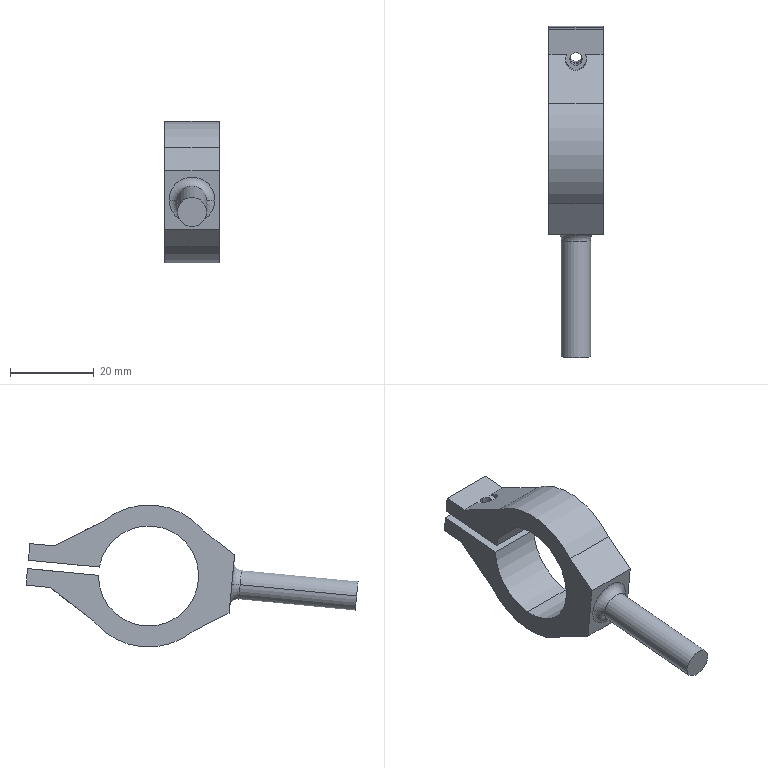Component | SolidWorks | Sleeve(Modified)-1 | 1 solid | 31 faces | box 13 x 79.45 x 34 mm | volume 9617 mm3 | cylinder 15 | plane 14 | torus 2 | commonest cylinder face diameters 3 x4 5 x3 34 x3 24 x3 7 x2 | material Plain Carbon Steel
build123d program:
from build123d import *

# Parameters (mm, degrees)
BOSS_EXTRUDE1_DEPTH      = 6.5
BOSS_EXTRUDE1_DEPTH_BACK = 6.5
SKETCH2_R                = 1.5
CUT_EXTRUDE1_DEPTH       = 37.976
SKETCH3_R                = 3.5
BOSS_EXTRUDE2_DEPTH      = 30
FILLET3_R                = 2
SKETCH4_R                = 2.5
CUT_EXTRUDE2_DEPTH       = 10


with BuildPart() as part:
    # Sketch1 → Boss-Extrude1 (new, two sides: drawn at the far end of the back side and taken through both)
    with BuildSketch(Plane.XY.offset(-BOSS_EXTRUDE1_DEPTH_BACK)):
        with BuildLine():
            Line((-1, 11.958), (-1, 29))
            Line((-1, 29), (-5, 29))
            Line((-5, 29), (-5, 23.19))
            Line((-5, 23.19), (-11.97, 12.071))
            ThreePointArc((-11.97, 12.071), (-17, 0), (-11.97, -12.071))
            Line((-11.97, -12.071), (-7, -20))
            Line((-7, -20), (7, -20))
            Line((7, -20), (11.97, -12.071))
            ThreePointArc((11.97, -12.071), (17, 0), (11.97, 12.071))
            Line((11.97, 12.071), (5, 23.19))
            Line((5, 23.19), (5, 29))
            Line((5, 29), (1, 29))
            Line((1, 29), (1, 11.958))
            ThreePointArc((1, 11.958), (0, -12), (-1, 11.958))
        make_face()
    extrude(amount=BOSS_EXTRUDE1_DEPTH + BOSS_EXTRUDE1_DEPTH_BACK)

    # Sketch2 → Cut-Extrude1 (cut, through all)
    with BuildSketch(Plane.ZY.offset(5)):
        with Locations(Location((0, 22, 0), (0, 0, 270))):
            Circle(SKETCH2_R)
    extrude(amount=-CUT_EXTRUDE1_DEPTH, mode=Mode.SUBTRACT)

    # Sketch3 → Boss-Extrude2 (add)
    with BuildSketch(Plane.XZ.offset(20)):
        with Locations(Location((0, 0, 0), (0, 0, 270))):
            Circle(SKETCH3_R)
    extrude(amount=BOSS_EXTRUDE2_DEPTH)

    # Fillet3
    fillet3_edges = [part.edges().sort_by_distance(p)[0] for p in [
        (0, -20, 3.5),
    ]]
    fillet(fillet3_edges, radius=FILLET3_R)

    # Sketch4 → Cut-Extrude2 (cut)
    with BuildSketch(Plane.ZY.offset(5)):
        with Locations((0, 22)):
            Circle(SKETCH4_R)
    cut_extrude2 = extrude(amount=CUT_EXTRUDE2_DEPTH, mode=Mode.SUBTRACT)

    # Mirror1: Cut-Extrude2 across plane
    add(cut_extrude2.mirror(Plane(origin=(0, 0, 0), x_dir=(0, 0, 1), z_dir=(1, 0, 0))), mode=Mode.SUBTRACT)


solid = part.part

# Placed as in the assembly
solid = solid.moved(Location((182.562, 15.115, 349), (5.48, -90, 0)))
STEP:
#1=CARTESIAN_POINT('',(7.274,1.523,13.631));
#2=VERTEX_POINT('',#1);
#3=CARTESIAN_POINT('',(7.187,1.387,13.527));
#4=VERTEX_POINT('',#3);
#5=CARTESIAN_POINT('',(7.274,1.523,13.631));
#6=CARTESIAN_POINT('',(7.314,1.454,13.579));
#7=CARTESIAN_POINT('',(7.271,1.387,13.527));
#8=CARTESIAN_POINT('',(7.187,1.387,13.527));
#9=(BOUNDED_CURVE()B_SPLINE_CURVE(3,(#5,#6,#7,#8),.UNSPECIFIED.,.F.,.F.)B_SPLINE_CURVE_WITH_KNOTS((4,4),(1.074,3.142),.UNSPECIFIED.)CURVE()GEOMETRIC_REPRESENTATION_ITEM()RATIONAL_B_SPLINE_CURVE((1.,0.6745,0.6745,1.))REPRESENTATION_ITEM(''));
#10=EDGE_CURVE('',#2,#4,#9,.T.);
#11=ORIENTED_EDGE('',*,*,#10,.T.);
#12=CARTESIAN_POINT('',(7.187,1.378,13.618));
#13=VERTEX_POINT('',#12);
#14=CARTESIAN_POINT('',(7.187,1.416,13.226));
#15=DIRECTION('',(0.,-0.09551,0.9954));
#16=VECTOR('',#15,39.37);
#17=LINE('',#14,#16);
#18=EDGE_CURVE('',#4,#13,#17,.T.);
#19=ORIENTED_EDGE('',*,*,#18,.T.);
#20=CARTESIAN_POINT('',(7.187,1.476,13.627));
#21=DIRECTION('',(0.,-0.09551,0.9954));
#22=DIRECTION('',(0.,-0.9954,-0.09551));
#23=AXIS2_PLACEMENT_3D('',#20,#21,#22);
#24=CIRCLE('',#23,0.09843);
#25=EDGE_CURVE('',#13,#2,#24,.T.);
#26=ORIENTED_EDGE('',*,*,#25,.T.);
#27=EDGE_LOOP('',(#11,#19,#26));
#28=FACE_OUTER_BOUND('',#27,.T.);
#29=CARTESIAN_POINT('',(7.187,1.514,13.235));
#30=DIRECTION('',(0.,-0.09551,0.9954));
#31=DIRECTION('',(0.,-0.9954,-0.09551));
#32=AXIS2_PLACEMENT_3D('',#29,#30,#31);
#33=CYLINDRICAL_SURFACE('',#32,0.09843);
#34=ADVANCED_FACE('',(#28),#33,.F.);
#35=CARTESIAN_POINT('',(7.05,-1.364,13.552));
#36=VERTEX_POINT('',#35);
#37=CARTESIAN_POINT('',(7.325,-1.364,13.552));
#38=VERTEX_POINT('',#37);
#39=CARTESIAN_POINT('',(7.187,-1.364,13.552));
#40=DIRECTION('',(0.,-0.9954,-0.09551));
#41=DIRECTION('',(-1.,0.,0.));
#42=AXIS2_PLACEMENT_3D('',#39,#40,#41);
#43=CIRCLE('',#42,0.1378);
#44=EDGE_CURVE('',#36,#38,#43,.T.);
#45=ORIENTED_EDGE('',*,*,#44,.F.);
#46=CARTESIAN_POINT('',(7.05,-0.2671,13.657));
#47=VERTEX_POINT('',#46);
#48=CARTESIAN_POINT('',(7.05,-1.364,13.552));
#49=DIRECTION('',(0.,0.9954,0.09551));
#50=VECTOR('',#49,39.37);
#51=LINE('',#48,#50);
#52=EDGE_CURVE('',#36,#47,#51,.T.);
#53=ORIENTED_EDGE('',*,*,#52,.T.);
#54=CARTESIAN_POINT('',(7.325,-0.2671,13.657));
#55=VERTEX_POINT('',#54);
#56=CARTESIAN_POINT('',(7.187,-0.2671,13.657));
#57=DIRECTION('',(0.,-0.9954,-0.09551));
#58=DIRECTION('',(-1.,0.,0.));
#59=AXIS2_PLACEMENT_3D('',#56,#57,#58);
#60=CIRCLE('',#59,0.1378);
#61=EDGE_CURVE('',#47,#55,#60,.T.);
#62=ORIENTED_EDGE('',*,*,#61,.T.);
#63=CARTESIAN_POINT('',(7.325,-1.364,13.552));
#64=DIRECTION('',(0.,0.9954,0.09551));
#65=VECTOR('',#64,39.37);
#66=LINE('',#63,#65);
#67=EDGE_CURVE('',#38,#55,#66,.T.);
#68=ORIENTED_EDGE('',*,*,#67,.F.);
#69=EDGE_LOOP('',(#45,#53,#62,#68));
#70=FACE_OUTER_BOUND('',#69,.T.);
#71=CARTESIAN_POINT('',(7.187,-1.364,13.552));
#72=DIRECTION('',(0.,0.9954,0.09551));
#73=DIRECTION('',(1.,0.,0.));
#74=AXIS2_PLACEMENT_3D('',#71,#72,#73);
#75=CYLINDRICAL_SURFACE('',#74,0.1378);
#76=ADVANCED_FACE('',(#70),#75,.T.);
#77=CARTESIAN_POINT('',(7.187,1.395,13.856));
#78=VERTEX_POINT('',#77);
#79=CARTESIAN_POINT('',(7.187,1.512,13.868));
#80=VERTEX_POINT('',#79);
#81=CARTESIAN_POINT('',(7.187,1.454,13.862));
#82=DIRECTION('',(0.,0.09551,-0.9954));
#83=DIRECTION('',(0.,0.9954,0.09551));
#84=AXIS2_PLACEMENT_3D('',#81,#82,#83);
#85=CIRCLE('',#84,0.05906);
#86=EDGE_CURVE('',#78,#80,#85,.T.);
#87=ORIENTED_EDGE('',*,*,#86,.T.);
#88=CARTESIAN_POINT('',(7.187,1.497,14.024));
#89=VERTEX_POINT('',#88);
#90=CARTESIAN_POINT('',(7.187,1.58,13.162));
#91=DIRECTION('',(0.,-0.09551,0.9954));
#92=VECTOR('',#91,39.37);
#93=LINE('',#90,#92);
#94=EDGE_CURVE('',#80,#89,#93,.T.);
#95=ORIENTED_EDGE('',*,*,#94,.T.);
#96=CARTESIAN_POINT('',(7.187,1.38,14.013));
#97=VERTEX_POINT('',#96);
#98=CARTESIAN_POINT('',(7.187,1.438,14.019));
#99=DIRECTION('',(0.,-0.09551,0.9954));
#100=DIRECTION('',(0.,-0.9954,-0.09551));
#101=AXIS2_PLACEMENT_3D('',#98,#99,#100);
#102=CIRCLE('',#101,0.05906);
#103=EDGE_CURVE('',#89,#97,#102,.T.);
#104=ORIENTED_EDGE('',*,*,#103,.T.);
#105=CARTESIAN_POINT('',(7.187,1.462,13.151));
#106=DIRECTION('',(0.,-0.09551,0.9954));
#107=VECTOR('',#106,39.37);
#108=LINE('',#105,#107);
#109=EDGE_CURVE('',#78,#97,#108,.T.);
#110=ORIENTED_EDGE('',*,*,#109,.F.);
#111=EDGE_LOOP('',(#87,#95,#104,#110));
#112=FACE_OUTER_BOUND('',#111,.T.);
#113=CARTESIAN_POINT('',(7.187,1.521,13.157));
#114=DIRECTION('',(0.,-0.09551,0.9954));
#115=DIRECTION('',(0.,-0.9954,-0.09551));
#116=AXIS2_PLACEMENT_3D('',#113,#114,#115);
#117=CYLINDRICAL_SURFACE('',#116,0.05906);
#118=ADVANCED_FACE('',(#112),#117,.F.);
#119=CARTESIAN_POINT('',(6.932,0.1671,13.226));
#120=VERTEX_POINT('',#119);
#121=CARTESIAN_POINT('',(6.932,0.659,13.074));
#122=VERTEX_POINT('',#121);
#123=CARTESIAN_POINT('',(6.932,0.5951,13.74));
#124=DIRECTION('',(1.,0.,0.));
#125=DIRECTION('',(0.,0.09551,-0.9954));
#126=AXIS2_PLACEMENT_3D('',#123,#124,#125);
#127=CIRCLE('',#126,0.6693);
#128=EDGE_CURVE('',#120,#122,#127,.T.);
#129=ORIENTED_EDGE('',*,*,#128,.T.);
#130=CARTESIAN_POINT('',(7.443,0.659,13.074));
#131=VERTEX_POINT('',#130);
#132=CARTESIAN_POINT('',(6.932,0.659,13.074));
#133=DIRECTION('',(1.,0.,0.));
#134=VECTOR('',#133,39.37);
#135=LINE('',#132,#134);
#136=EDGE_CURVE('',#122,#131,#135,.T.);
#137=ORIENTED_EDGE('',*,*,#136,.T.);
#138=CARTESIAN_POINT('',(7.443,0.1671,13.226));
#139=VERTEX_POINT('',#138);
#140=CARTESIAN_POINT('',(7.443,0.5951,13.74));
#141=DIRECTION('',(1.,0.,0.));
#142=DIRECTION('',(0.,0.09551,-0.9954));
#143=AXIS2_PLACEMENT_3D('',#140,#141,#142);
#144=CIRCLE('',#143,0.6693);
#145=EDGE_CURVE('',#139,#131,#144,.T.);
#146=ORIENTED_EDGE('',*,*,#145,.F.);
#147=CARTESIAN_POINT('',(6.932,0.1671,13.226));
#148=DIRECTION('',(1.,0.,0.));
#149=VECTOR('',#148,39.37);
#150=LINE('',#147,#149);
#151=EDGE_CURVE('',#120,#139,#150,.T.);
#152=ORIENTED_EDGE('',*,*,#151,.F.);
#153=EDGE_LOOP('',(#129,#137,#146,#152));
#154=FACE_OUTER_BOUND('',#153,.T.);
#155=CARTESIAN_POINT('',(6.932,0.5951,13.74));
#156=DIRECTION('',(1.,0.,0.));
#157=DIRECTION('',(0.,0.09551,-0.9954));
#158=AXIS2_PLACEMENT_3D('',#155,#156,#157);
#159=CYLINDRICAL_SURFACE('',#158,0.6693);
#160=ADVANCED_FACE('',(#154),#159,.T.);
#161=CARTESIAN_POINT('',(6.932,0.6402,13.27));
#162=VERTEX_POINT('',#161);
#163=CARTESIAN_POINT('',(6.932,0.55,14.21));
#164=VERTEX_POINT('',#163);
#165=CARTESIAN_POINT('',(6.932,0.5951,13.74));
#166=DIRECTION('',(-1.,0.,0.));
#167=DIRECTION('',(0.,0.09551,-0.9954));
#168=AXIS2_PLACEMENT_3D('',#165,#166,#167);
#169=CIRCLE('',#168,0.4724);
#170=EDGE_CURVE('',#162,#164,#169,.T.);
#171=ORIENTED_EDGE('',*,*,#170,.T.);
#172=CARTESIAN_POINT('',(7.443,0.55,14.21));
#173=VERTEX_POINT('',#172);
#174=CARTESIAN_POINT('',(6.932,0.55,14.21));
#175=DIRECTION('',(1.,0.,0.));
#176=VECTOR('',#175,39.37);
#177=LINE('',#174,#176);
#178=EDGE_CURVE('',#164,#173,#177,.T.);
#179=ORIENTED_EDGE('',*,*,#178,.T.);
#180=CARTESIAN_POINT('',(7.443,0.6402,13.27));
#181=VERTEX_POINT('',#180);
#182=CARTESIAN_POINT('',(7.443,0.5951,13.74));
#183=DIRECTION('',(-1.,0.,0.));
#184=DIRECTION('',(0.,0.09551,-0.9954));
#185=AXIS2_PLACEMENT_3D('',#182,#183,#184);
#186=CIRCLE('',#185,0.4724);
#187=EDGE_CURVE('',#181,#173,#186,.T.);
#188=ORIENTED_EDGE('',*,*,#187,.F.);
#189=CARTESIAN_POINT('',(6.932,0.6402,13.27));
#190=DIRECTION('',(1.,0.,0.));
#191=VECTOR('',#190,39.37);
#192=LINE('',#189,#191);
#193=EDGE_CURVE('',#162,#181,#192,.T.);
#194=ORIENTED_EDGE('',*,*,#193,.F.);
#195=EDGE_LOOP('',(#171,#179,#188,#194));
#196=FACE_OUTER_BOUND('',#195,.T.);
#197=CARTESIAN_POINT('',(6.932,0.5951,13.74));
#198=DIRECTION('',(1.,0.,0.));
#199=DIRECTION('',(0.,0.09551,-0.9954));
#200=AXIS2_PLACEMENT_3D('',#197,#198,#199);
#201=CYLINDRICAL_SURFACE('',#200,0.4724);
#202=ADVANCED_FACE('',(#196),#201,.F.);
#203=CARTESIAN_POINT('',(6.932,1.068,13.746));
#204=VERTEX_POINT('',#203);
#205=CARTESIAN_POINT('',(6.932,0.5951,13.74));
#206=DIRECTION('',(-1.,0.,0.));
#207=DIRECTION('',(0.,0.09551,-0.9954));
#208=AXIS2_PLACEMENT_3D('',#205,#206,#207);
#209=CIRCLE('',#208,0.4724);
#210=EDGE_CURVE('',#204,#162,#209,.T.);
#211=ORIENTED_EDGE('',*,*,#210,.T.);
#212=ORIENTED_EDGE('',*,*,#193,.T.);
#213=CARTESIAN_POINT('',(7.443,1.068,13.746));
#214=VERTEX_POINT('',#213);
#215=CARTESIAN_POINT('',(7.443,0.5951,13.74));
#216=DIRECTION('',(-1.,0.,0.));
#217=DIRECTION('',(0.,0.09551,-0.9954));
#218=AXIS2_PLACEMENT_3D('',#215,#216,#217);
#219=CIRCLE('',#218,0.4724);
#220=EDGE_CURVE('',#214,#181,#219,.T.);
#221=ORIENTED_EDGE('',*,*,#220,.F.);
#222=CARTESIAN_POINT('',(6.932,1.068,13.746));
#223=DIRECTION('',(1.,0.,0.));
#224=VECTOR('',#223,39.37);
#225=LINE('',#222,#224);
#226=EDGE_CURVE('',#204,#214,#225,.T.);
#227=ORIENTED_EDGE('',*,*,#226,.F.);
#228=EDGE_LOOP('',(#211,#212,#221,#227));
#229=FACE_OUTER_BOUND('',#228,.T.);
#230=CARTESIAN_POINT('',(6.932,0.5951,13.74));
#231=DIRECTION('',(1.,0.,0.));
#232=DIRECTION('',(0.,0.09551,-0.9954));
#233=AXIS2_PLACEMENT_3D('',#230,#231,#232);
#234=CYLINDRICAL_SURFACE('',#233,0.4724);
#235=ADVANCED_FACE('',(#229),#234,.F.);
#236=CARTESIAN_POINT('',(7.187,-0.2671,13.657));
#237=DIRECTION('',(0.,-0.9954,-0.09551));
#238=DIRECTION('',(-1.,0.,0.));
#239=AXIS2_PLACEMENT_3D('',#236,#237,#238);
#240=CIRCLE('',#239,0.1378);
#241=EDGE_CURVE('',#55,#47,#240,.T.);
#242=ORIENTED_EDGE('',*,*,#241,.F.);
#243=CARTESIAN_POINT('',(7.404,-0.1887,13.665));
#244=VERTEX_POINT('',#243);
#245=CARTESIAN_POINT('',(7.404,-0.2671,13.657));
#246=DIRECTION('',(-0.,0.09551,-0.9954));
#247=DIRECTION('',(0.,0.9954,0.09551));
#248=AXIS2_PLACEMENT_3D('',#245,#246,#247);
#249=CIRCLE('',#248,0.07874);
#250=EDGE_CURVE('',#55,#244,#249,.T.);
#251=ORIENTED_EDGE('',*,*,#250,.T.);
#252=CARTESIAN_POINT('',(6.971,-0.1887,13.665));
#253=VERTEX_POINT('',#252);
#254=CARTESIAN_POINT('',(7.187,-0.1887,13.665));
#255=DIRECTION('',(0.,0.9954,0.09551));
#256=DIRECTION('',(-1.,0.,0.));
#257=AXIS2_PLACEMENT_3D('',#254,#255,#256);
#258=CIRCLE('',#257,0.2165);
#259=EDGE_CURVE('',#253,#244,#258,.T.);
#260=ORIENTED_EDGE('',*,*,#259,.F.);
#261=CARTESIAN_POINT('',(6.971,-0.2671,13.657));
#262=DIRECTION('',(0.,-0.09551,0.9954));
#263=DIRECTION('',(0.,-0.9954,-0.09551));
#264=AXIS2_PLACEMENT_3D('',#261,#262,#263);
#265=CIRCLE('',#264,0.07874);
#266=EDGE_CURVE('',#47,#253,#265,.T.);
#267=ORIENTED_EDGE('',*,*,#266,.F.);
#268=EDGE_LOOP('',(#242,#251,#260,#267));
#269=FACE_OUTER_BOUND('',#268,.T.);
#270=CARTESIAN_POINT('',(7.187,-0.2671,13.657));
#271=DIRECTION('',(0.,-0.9954,-0.09551));
#272=DIRECTION('',(-1.,0.,0.));
#273=AXIS2_PLACEMENT_3D('',#270,#271,#272);
#274=TOROIDAL_SURFACE('',#273,0.2165,0.07874);
#275=ADVANCED_FACE('',(#269),#274,.F.);
#276=CARTESIAN_POINT('',(7.187,1.417,13.621));
#277=VERTEX_POINT('',#276);
#278=CARTESIAN_POINT('',(7.187,1.535,13.633));
#279=VERTEX_POINT('',#278);
#280=CARTESIAN_POINT('',(7.187,1.476,13.627));
#281=DIRECTION('',(0.,0.09551,-0.9954));
#282=DIRECTION('',(-1.,0.,0.));
#283=AXIS2_PLACEMENT_3D('',#280,#281,#282);
#284=CIRCLE('',#283,0.05906);
#285=EDGE_CURVE('',#277,#279,#284,.T.);
#286=ORIENTED_EDGE('',*,*,#285,.T.);
#287=CARTESIAN_POINT('',(7.187,1.52,13.789));
#288=VERTEX_POINT('',#287);
#289=CARTESIAN_POINT('',(7.187,1.58,13.162));
#290=DIRECTION('',(0.,-0.09551,0.9954));
#291=VECTOR('',#290,39.37);
#292=LINE('',#289,#291);
#293=EDGE_CURVE('',#279,#288,#292,.T.);
#294=ORIENTED_EDGE('',*,*,#293,.T.);
#295=CARTESIAN_POINT('',(7.187,1.402,13.778));
#296=VERTEX_POINT('',#295);
#297=CARTESIAN_POINT('',(7.187,1.461,13.784));
#298=DIRECTION('',(0.,-0.09551,0.9954));
#299=DIRECTION('',(0.,-0.9954,-0.09551));
#300=AXIS2_PLACEMENT_3D('',#297,#298,#299);
#301=CIRCLE('',#300,0.05906);
#302=EDGE_CURVE('',#288,#296,#301,.T.);
#303=ORIENTED_EDGE('',*,*,#302,.T.);
#304=CARTESIAN_POINT('',(7.187,1.462,13.151));
#305=DIRECTION('',(0.,-0.09551,0.9954));
#306=VECTOR('',#305,39.37);
#307=LINE('',#304,#306);
#308=EDGE_CURVE('',#277,#296,#307,.T.);
#309=ORIENTED_EDGE('',*,*,#308,.F.);
#310=EDGE_LOOP('',(#286,#294,#303,#309));
#311=FACE_OUTER_BOUND('',#310,.T.);
#312=CARTESIAN_POINT('',(7.187,1.521,13.157));
#313=DIRECTION('',(0.,-0.09551,0.9954));
#314=DIRECTION('',(0.,-0.9954,-0.09551));
#315=AXIS2_PLACEMENT_3D('',#312,#313,#314);
#316=CYLINDRICAL_SURFACE('',#315,0.05906);
#317=ADVANCED_FACE('',(#311),#316,.F.);
#318=ORIENTED_EDGE('',*,*,#293,.F.);
#319=CARTESIAN_POINT('',(7.187,1.476,13.627));
#320=DIRECTION('',(0.,0.09551,-0.9954));
#321=DIRECTION('',(-1.,0.,0.));
#322=AXIS2_PLACEMENT_3D('',#319,#320,#321);
#323=CIRCLE('',#322,0.05906);
#324=EDGE_CURVE('',#279,#277,#323,.T.);
#325=ORIENTED_EDGE('',*,*,#324,.T.);
#326=ORIENTED_EDGE('',*,*,#308,.T.);
#327=CARTESIAN_POINT('',(7.187,1.461,13.784));
#328=DIRECTION('',(0.,-0.09551,0.9954));
#329=DIRECTION('',(0.,-0.9954,-0.09551));
#330=AXIS2_PLACEMENT_3D('',#327,#328,#329);
#331=CIRCLE('',#330,0.05906);
#332=EDGE_CURVE('',#296,#288,#331,.T.);
#333=ORIENTED_EDGE('',*,*,#332,.T.);
#334=EDGE_LOOP('',(#318,#325,#326,#333));
#335=FACE_OUTER_BOUND('',#334,.T.);
#336=CARTESIAN_POINT('',(7.187,1.521,13.157));
#337=DIRECTION('',(0.,-0.09551,0.9954));
#338=DIRECTION('',(0.,-0.9954,-0.09551));
#339=AXIS2_PLACEMENT_3D('',#336,#337,#338);
#340=CYLINDRICAL_SURFACE('',#339,0.05906);
#341=ADVANCED_FACE('',(#335),#340,.F.);
#342=CARTESIAN_POINT('',(7.274,1.485,14.023));
#343=VERTEX_POINT('',#342);
#344=CARTESIAN_POINT('',(7.443,1.485,14.023));
#345=VERTEX_POINT('',#344);
#346=CARTESIAN_POINT('',(6.932,1.485,14.023));
#347=DIRECTION('',(1.,0.,0.));
#348=VECTOR('',#347,39.37);
#349=LINE('',#346,#348);
#350=EDGE_CURVE('',#343,#345,#349,.T.);
#351=ORIENTED_EDGE('',*,*,#350,.F.);
#352=CARTESIAN_POINT('',(7.101,1.485,14.023));
#353=VERTEX_POINT('',#352);
#354=CARTESIAN_POINT('',(7.274,1.485,14.023));
#355=CARTESIAN_POINT('',(7.314,1.408,14.062));
#356=CARTESIAN_POINT('',(7.271,1.332,14.1));
#357=CARTESIAN_POINT('',(7.187,1.332,14.1));
#358=CARTESIAN_POINT('',(7.104,1.332,14.1));
#359=CARTESIAN_POINT('',(7.061,1.408,14.062));
#360=CARTESIAN_POINT('',(7.101,1.485,14.023));
#361=(BOUNDED_CURVE()B_SPLINE_CURVE(3,(#354,#355,#356,#357,#358,#359,#360),.UNSPECIFIED.,.F.,.F.)B_SPLINE_CURVE_WITH_KNOTS((4,3,4),(1.074,3.142,5.209),.UNSPECIFIED.)CURVE()GEOMETRIC_REPRESENTATION_ITEM()RATIONAL_B_SPLINE_CURVE((1.,0.6745,0.6745,1.,0.6745,0.6745,1.))REPRESENTATION_ITEM(''));
#362=EDGE_CURVE('',#343,#353,#361,.T.);
#363=ORIENTED_EDGE('',*,*,#362,.T.);
#364=CARTESIAN_POINT('',(6.932,1.485,14.023));
#365=VERTEX_POINT('',#364);
#366=CARTESIAN_POINT('',(6.932,1.485,14.023));
#367=DIRECTION('',(1.,0.,0.));
#368=VECTOR('',#367,39.37);
#369=LINE('',#366,#368);
#370=EDGE_CURVE('',#365,#353,#369,.T.);
#371=ORIENTED_EDGE('',*,*,#370,.F.);
#372=CARTESIAN_POINT('',(6.932,1.023,14.255));
#373=VERTEX_POINT('',#372);
#374=CARTESIAN_POINT('',(6.932,1.023,14.255));
#375=DIRECTION('',(0.,-0.8941,0.4478));
#376=VECTOR('',#375,39.37);
#377=LINE('',#374,#376);
#378=EDGE_CURVE('',#365,#373,#377,.T.);
#379=ORIENTED_EDGE('',*,*,#378,.T.);
#380=CARTESIAN_POINT('',(7.443,1.023,14.255));
#381=VERTEX_POINT('',#380);
#382=CARTESIAN_POINT('',(6.932,1.023,14.255));
#383=DIRECTION('',(1.,0.,0.));
#384=VECTOR('',#383,39.37);
#385=LINE('',#382,#384);
#386=EDGE_CURVE('',#373,#381,#385,.T.);
#387=ORIENTED_EDGE('',*,*,#386,.T.);
#388=CARTESIAN_POINT('',(7.443,1.023,14.255));
#389=DIRECTION('',(0.,-0.8941,0.4478));
#390=VECTOR('',#389,39.37);
#391=LINE('',#388,#390);
#392=EDGE_CURVE('',#345,#381,#391,.T.);
#393=ORIENTED_EDGE('',*,*,#392,.F.);
#394=EDGE_LOOP('',(#351,#363,#371,#379,#387,#393));
#395=FACE_OUTER_BOUND('',#394,.T.);
#396=CARTESIAN_POINT('',(6.932,1.023,14.255));
#397=DIRECTION('',(0.,0.4478,0.8941));
#398=DIRECTION('',(0.,-0.8941,0.4478));
#399=AXIS2_PLACEMENT_3D('',#396,#397,#398);
#400=PLANE('',#399);
#401=ADVANCED_FACE('',(#395),#400,.T.);
#402=ORIENTED_EDGE('',*,*,#250,.F.);
#403=ORIENTED_EDGE('',*,*,#61,.F.);
#404=ORIENTED_EDGE('',*,*,#266,.T.);
#405=CARTESIAN_POINT('',(7.187,-0.1887,13.665));
#406=DIRECTION('',(0.,0.9954,0.09551));
#407=DIRECTION('',(-1.,0.,0.));
#408=AXIS2_PLACEMENT_3D('',#405,#406,#407);
#409=CIRCLE('',#408,0.2165);
#410=EDGE_CURVE('',#244,#253,#409,.T.);
#411=ORIENTED_EDGE('',*,*,#410,.F.);
#412=EDGE_LOOP('',(#402,#403,#404,#411));
#413=FACE_OUTER_BOUND('',#412,.T.);
#414=CARTESIAN_POINT('',(7.187,-0.2671,13.657));
#415=DIRECTION('',(0.,-0.9954,-0.09551));
#416=DIRECTION('',(-1.,0.,0.));
#417=AXIS2_PLACEMENT_3D('',#414,#415,#416);
#418=TOROIDAL_SURFACE('',#417,0.2165,0.07874);
#419=ADVANCED_FACE('',(#413),#418,.F.);
#420=ORIENTED_EDGE('',*,*,#259,.T.);
#421=ORIENTED_EDGE('',*,*,#410,.T.);
#422=EDGE_LOOP('',(#420,#421));
#423=FACE_BOUND('',#422,.T.);
#424=CARTESIAN_POINT('',(6.932,-0.1624,13.391));
#425=VERTEX_POINT('',#424);
#426=CARTESIAN_POINT('',(7.443,-0.1624,13.391));
#427=VERTEX_POINT('',#426);
#428=CARTESIAN_POINT('',(6.932,-0.1624,13.391));
#429=DIRECTION('',(1.,0.,0.));
#430=VECTOR('',#429,39.37);
#431=LINE('',#428,#430);
#432=EDGE_CURVE('',#425,#427,#431,.T.);
#433=ORIENTED_EDGE('',*,*,#432,.T.);
#434=CARTESIAN_POINT('',(7.443,-0.215,13.939));
#435=VERTEX_POINT('',#434);
#436=CARTESIAN_POINT('',(7.443,-0.215,13.939));
#437=DIRECTION('',(0.,0.09551,-0.9954));
#438=VECTOR('',#437,39.37);
#439=LINE('',#436,#438);
#440=EDGE_CURVE('',#435,#427,#439,.T.);
#441=ORIENTED_EDGE('',*,*,#440,.F.);
#442=CARTESIAN_POINT('',(6.932,-0.215,13.939));
#443=VERTEX_POINT('',#442);
#444=CARTESIAN_POINT('',(6.932,-0.215,13.939));
#445=DIRECTION('',(1.,0.,0.));
#446=VECTOR('',#445,39.37);
#447=LINE('',#444,#446);
#448=EDGE_CURVE('',#443,#435,#447,.T.);
#449=ORIENTED_EDGE('',*,*,#448,.F.);
#450=CARTESIAN_POINT('',(6.932,-0.215,13.939));
#451=DIRECTION('',(0.,0.09551,-0.9954));
#452=VECTOR('',#451,39.37);
#453=LINE('',#450,#452);
#454=EDGE_CURVE('',#443,#425,#453,.T.);
#455=ORIENTED_EDGE('',*,*,#454,.T.);
#456=EDGE_LOOP('',(#433,#441,#449,#455));
#457=FACE_OUTER_BOUND('',#456,.T.);
#458=CARTESIAN_POINT('',(6.932,-0.215,13.939));
#459=DIRECTION('',(0.,-0.9954,-0.09551));
#460=DIRECTION('',(-1.,0.,0.));
#461=AXIS2_PLACEMENT_3D('',#458,#459,#460);
#462=PLANE('',#461);
#463=ADVANCED_FACE('',(#423,#457),#462,.T.);
#464=CARTESIAN_POINT('',(6.932,0.07703,14.164));
#465=VERTEX_POINT('',#464);
#466=CARTESIAN_POINT('',(7.443,0.07703,14.164));
#467=VERTEX_POINT('',#466);
#468=CARTESIAN_POINT('',(6.932,0.07703,14.164));
#469=DIRECTION('',(1.,0.,0.));
#470=VECTOR('',#469,39.37);
#471=LINE('',#468,#470);
#472=EDGE_CURVE('',#465,#467,#471,.T.);
#473=ORIENTED_EDGE('',*,*,#472,.T.);
#474=CARTESIAN_POINT('',(7.443,0.5951,13.74));
#475=DIRECTION('',(1.,0.,0.));
#476=DIRECTION('',(0.,0.09551,-0.9954));
#477=AXIS2_PLACEMENT_3D('',#474,#475,#476);
#478=CIRCLE('',#477,0.6693);
#479=EDGE_CURVE('',#381,#467,#478,.T.);
#480=ORIENTED_EDGE('',*,*,#479,.F.);
#481=ORIENTED_EDGE('',*,*,#386,.F.);
#482=CARTESIAN_POINT('',(6.932,0.5951,13.74));
#483=DIRECTION('',(1.,0.,0.));
#484=DIRECTION('',(0.,0.09551,-0.9954));
#485=AXIS2_PLACEMENT_3D('',#482,#483,#484);
#486=CIRCLE('',#485,0.6693);
#487=EDGE_CURVE('',#373,#465,#486,.T.);
#488=ORIENTED_EDGE('',*,*,#487,.T.);
#489=EDGE_LOOP('',(#473,#480,#481,#488));
#490=FACE_OUTER_BOUND('',#489,.T.);
#491=CARTESIAN_POINT('',(6.932,0.5951,13.74));
#492=DIRECTION('',(1.,0.,0.));
#493=DIRECTION('',(0.,0.09551,-0.9954));
#494=AXIS2_PLACEMENT_3D('',#491,#492,#493);
#495=CYLINDRICAL_SURFACE('',#494,0.6693);
#496=ADVANCED_FACE('',(#490),#495,.T.);
#497=CARTESIAN_POINT('',(7.187,1.438,14.019));
#498=DIRECTION('',(0.,-0.09551,0.9954));
#499=DIRECTION('',(0.,-0.9954,-0.09551));
#500=AXIS2_PLACEMENT_3D('',#497,#498,#499);
#501=CIRCLE('',#500,0.05906);
#502=EDGE_CURVE('',#97,#89,#501,.T.);
#503=ORIENTED_EDGE('',*,*,#502,.F.);
#504=ORIENTED_EDGE('',*,*,#103,.F.);
#505=EDGE_LOOP('',(#503,#504));
#506=FACE_BOUND('',#505,.T.);
#507=ORIENTED_EDGE('',*,*,#370,.T.);
#508=CARTESIAN_POINT('',(7.187,1.438,14.019));
#509=DIRECTION('',(0.,-0.09551,0.9954));
#510=DIRECTION('',(0.,-0.9954,-0.09551));
#511=AXIS2_PLACEMENT_3D('',#508,#509,#510);
#512=CIRCLE('',#511,0.09843);
#513=EDGE_CURVE('',#353,#343,#512,.T.);
#514=ORIENTED_EDGE('',*,*,#513,.T.);
#515=ORIENTED_EDGE('',*,*,#350,.T.);
#516=CARTESIAN_POINT('',(7.443,1.713,14.045));
#517=VERTEX_POINT('',#516);
#518=CARTESIAN_POINT('',(7.443,1.713,14.045));
#519=DIRECTION('',(0.,-0.9954,-0.09551));
#520=VECTOR('',#519,39.37);
#521=LINE('',#518,#520);
#522=EDGE_CURVE('',#517,#345,#521,.T.);
#523=ORIENTED_EDGE('',*,*,#522,.F.);
#524=CARTESIAN_POINT('',(6.932,1.713,14.045));
#525=VERTEX_POINT('',#524);
#526=CARTESIAN_POINT('',(6.932,1.713,14.045));
#527=DIRECTION('',(1.,0.,0.));
#528=VECTOR('',#527,39.37);
#529=LINE('',#526,#528);
#530=EDGE_CURVE('',#525,#517,#529,.T.);
#531=ORIENTED_EDGE('',*,*,#530,.F.);
#532=CARTESIAN_POINT('',(6.932,1.713,14.045));
#533=DIRECTION('',(0.,-0.9954,-0.09551));
#534=VECTOR('',#533,39.37);
#535=LINE('',#532,#534);
#536=EDGE_CURVE('',#525,#365,#535,.T.);
#537=ORIENTED_EDGE('',*,*,#536,.T.);
#538=EDGE_LOOP('',(#507,#514,#515,#523,#531,#537));
#539=FACE_OUTER_BOUND('',#538,.T.);
#540=CARTESIAN_POINT('',(6.932,1.713,14.045));
#541=DIRECTION('',(0.,-0.09551,0.9954));
#542=DIRECTION('',(0.,-0.9954,-0.09551));
#543=AXIS2_PLACEMENT_3D('',#540,#541,#542);
#544=PLANE('',#543);
#545=ADVANCED_FACE('',(#506,#539),#544,.T.);
#546=ORIENTED_EDGE('',*,*,#530,.T.);
#547=CARTESIAN_POINT('',(7.443,1.728,13.888));
#548=VERTEX_POINT('',#547);
#549=CARTESIAN_POINT('',(7.443,1.728,13.888));
#550=DIRECTION('',(0.,-0.09551,0.9954));
#551=VECTOR('',#550,39.37);
#552=LINE('',#549,#551);
#553=EDGE_CURVE('',#548,#517,#552,.T.);
#554=ORIENTED_EDGE('',*,*,#553,.F.);
#555=CARTESIAN_POINT('',(6.932,1.728,13.888));
#556=VERTEX_POINT('',#555);
#557=CARTESIAN_POINT('',(6.932,1.728,13.888));
#558=DIRECTION('',(1.,0.,0.));
#559=VECTOR('',#558,39.37);
#560=LINE('',#557,#559);
#561=EDGE_CURVE('',#556,#548,#560,.T.);
#562=ORIENTED_EDGE('',*,*,#561,.F.);
#563=CARTESIAN_POINT('',(6.932,1.728,13.888));
#564=DIRECTION('',(0.,-0.09551,0.9954));
#565=VECTOR('',#564,39.37);
#566=LINE('',#563,#565);
#567=EDGE_CURVE('',#556,#525,#566,.T.);
#568=ORIENTED_EDGE('',*,*,#567,.T.);
#569=EDGE_LOOP('',(#546,#554,#562,#568));
#570=FACE_OUTER_BOUND('',#569,.T.);
#571=CARTESIAN_POINT('',(6.932,1.728,13.888));
#572=DIRECTION('',(0.,0.9954,0.09551));
#573=DIRECTION('',(1.,0.,0.));
#574=AXIS2_PLACEMENT_3D('',#571,#572,#573);
#575=PLANE('',#574);
#576=ADVANCED_FACE('',(#570),#575,.T.);
#577=ORIENTED_EDGE('',*,*,#86,.F.);
#578=CARTESIAN_POINT('',(7.187,1.454,13.862));
#579=DIRECTION('',(0.,0.09551,-0.9954));
#580=DIRECTION('',(0.,0.9954,0.09551));
#581=AXIS2_PLACEMENT_3D('',#578,#579,#580);
#582=CIRCLE('',#581,0.05906);
#583=EDGE_CURVE('',#80,#78,#582,.T.);
#584=ORIENTED_EDGE('',*,*,#583,.F.);
#585=EDGE_LOOP('',(#577,#584));
#586=FACE_BOUND('',#585,.T.);
#587=ORIENTED_EDGE('',*,*,#561,.T.);
#588=CARTESIAN_POINT('',(7.443,1.06,13.824));
#589=VERTEX_POINT('',#588);
#590=CARTESIAN_POINT('',(7.443,1.06,13.824));
#591=DIRECTION('',(0.,0.9954,0.09551));
#592=VECTOR('',#591,39.37);
#593=LINE('',#590,#592);
#594=EDGE_CURVE('',#589,#548,#593,.T.);
#595=ORIENTED_EDGE('',*,*,#594,.F.);
#596=CARTESIAN_POINT('',(6.932,1.06,13.824));
#597=VERTEX_POINT('',#596);
#598=CARTESIAN_POINT('',(6.932,1.06,13.824));
#599=DIRECTION('',(1.,0.,0.));
#600=VECTOR('',#599,39.37);
#601=LINE('',#598,#600);
#602=EDGE_CURVE('',#597,#589,#601,.T.);
#603=ORIENTED_EDGE('',*,*,#602,.F.);
#604=CARTESIAN_POINT('',(6.932,1.06,13.824));
#605=DIRECTION('',(0.,0.9954,0.09551));
#606=VECTOR('',#605,39.37);
#607=LINE('',#604,#606);
#608=EDGE_CURVE('',#597,#556,#607,.T.);
#609=ORIENTED_EDGE('',*,*,#608,.T.);
#610=EDGE_LOOP('',(#587,#595,#603,#609));
#611=FACE_OUTER_BOUND('',#610,.T.);
#612=CARTESIAN_POINT('',(6.932,1.06,13.824));
#613=DIRECTION('',(0.,0.09551,-0.9954));
#614=DIRECTION('',(0.,0.9954,0.09551));
#615=AXIS2_PLACEMENT_3D('',#612,#613,#614);
#616=PLANE('',#615);
#617=ADVANCED_FACE('',(#586,#611),#616,.T.);
#618=ORIENTED_EDGE('',*,*,#178,.F.);
#619=CARTESIAN_POINT('',(6.932,0.5951,13.74));
#620=DIRECTION('',(-1.,0.,0.));
#621=DIRECTION('',(0.,0.09551,-0.9954));
#622=AXIS2_PLACEMENT_3D('',#619,#620,#621);
#623=CIRCLE('',#622,0.4724);
#624=EDGE_CURVE('',#164,#597,#623,.T.);
#625=ORIENTED_EDGE('',*,*,#624,.T.);
#626=ORIENTED_EDGE('',*,*,#602,.T.);
#627=CARTESIAN_POINT('',(7.443,0.5951,13.74));
#628=DIRECTION('',(-1.,0.,0.));
#629=DIRECTION('',(0.,0.09551,-0.9954));
#630=AXIS2_PLACEMENT_3D('',#627,#628,#629);
#631=CIRCLE('',#630,0.4724);
#632=EDGE_CURVE('',#173,#589,#631,.T.);
#633=ORIENTED_EDGE('',*,*,#632,.F.);
#634=EDGE_LOOP('',(#618,#625,#626,#633));
#635=FACE_OUTER_BOUND('',#634,.T.);
#636=CARTESIAN_POINT('',(6.932,0.5951,13.74));
#637=DIRECTION('',(1.,0.,0.));
#638=DIRECTION('',(0.,0.09551,-0.9954));
#639=AXIS2_PLACEMENT_3D('',#636,#637,#638);
#640=CYLINDRICAL_SURFACE('',#639,0.4724);
#641=ADVANCED_FACE('',(#635),#640,.F.);
#642=ORIENTED_EDGE('',*,*,#332,.F.);
#643=ORIENTED_EDGE('',*,*,#302,.F.);
#644=EDGE_LOOP('',(#642,#643));
#645=FACE_BOUND('',#644,.T.);
#646=ORIENTED_EDGE('',*,*,#226,.T.);
#647=CARTESIAN_POINT('',(7.443,1.735,13.81));
#648=VERTEX_POINT('',#647);
#649=CARTESIAN_POINT('',(7.443,1.068,13.746));
#650=DIRECTION('',(0.,-0.9954,-0.09551));
#651=VECTOR('',#650,39.37);
#652=LINE('',#649,#651);
#653=EDGE_CURVE('',#648,#214,#652,.T.);
#654=ORIENTED_EDGE('',*,*,#653,.F.);
#655=CARTESIAN_POINT('',(6.932,1.735,13.81));
#656=VERTEX_POINT('',#655);
#657=CARTESIAN_POINT('',(6.932,1.735,13.81));
#658=DIRECTION('',(1.,0.,0.));
#659=VECTOR('',#658,39.37);
#660=LINE('',#657,#659);
#661=EDGE_CURVE('',#656,#648,#660,.T.);
#662=ORIENTED_EDGE('',*,*,#661,.F.);
#663=CARTESIAN_POINT('',(6.932,1.068,13.746));
#664=DIRECTION('',(0.,-0.9954,-0.09551));
#665=VECTOR('',#664,39.37);
#666=LINE('',#663,#665);
#667=EDGE_CURVE('',#656,#204,#666,.T.);
#668=ORIENTED_EDGE('',*,*,#667,.T.);
#669=EDGE_LOOP('',(#646,#654,#662,#668));
#670=FACE_OUTER_BOUND('',#669,.T.);
#671=CARTESIAN_POINT('',(6.932,1.068,13.746));
#672=DIRECTION('',(0.,-0.09551,0.9954));
#673=DIRECTION('',(0.,-0.9954,-0.09551));
#674=AXIS2_PLACEMENT_3D('',#671,#672,#673);
#675=PLANE('',#674);
#676=ADVANCED_FACE('',(#645,#670),#675,.T.);
#677=ORIENTED_EDGE('',*,*,#661,.T.);
#678=CARTESIAN_POINT('',(7.443,1.75,13.653));
#679=VERTEX_POINT('',#678);
#680=CARTESIAN_POINT('',(7.443,1.735,13.81));
#681=DIRECTION('',(0.,-0.09551,0.9954));
#682=VECTOR('',#681,39.37);
#683=LINE('',#680,#682);
#684=EDGE_CURVE('',#679,#648,#683,.T.);
#685=ORIENTED_EDGE('',*,*,#684,.F.);
#686=CARTESIAN_POINT('',(6.932,1.75,13.653));
#687=VERTEX_POINT('',#686);
#688=CARTESIAN_POINT('',(6.932,1.75,13.653));
#689=DIRECTION('',(1.,0.,0.));
#690=VECTOR('',#689,39.37);
#691=LINE('',#688,#690);
#692=EDGE_CURVE('',#687,#679,#691,.T.);
#693=ORIENTED_EDGE('',*,*,#692,.F.);
#694=CARTESIAN_POINT('',(6.932,1.735,13.81));
#695=DIRECTION('',(0.,-0.09551,0.9954));
#696=VECTOR('',#695,39.37);
#697=LINE('',#694,#696);
#698=EDGE_CURVE('',#687,#656,#697,.T.);
#699=ORIENTED_EDGE('',*,*,#698,.T.);
#700=EDGE_LOOP('',(#677,#685,#693,#699));
#701=FACE_OUTER_BOUND('',#700,.T.);
#702=CARTESIAN_POINT('',(6.932,1.735,13.81));
#703=DIRECTION('',(0.,0.9954,0.09551));
#704=DIRECTION('',(1.,0.,0.));
#705=AXIS2_PLACEMENT_3D('',#702,#703,#704);
#706=PLANE('',#705);
#707=ADVANCED_FACE('',(#701),#706,.T.);
#708=CARTESIAN_POINT('',(7.443,1.523,13.631));
#709=VERTEX_POINT('',#708);
#710=CARTESIAN_POINT('',(6.932,1.523,13.631));
#711=DIRECTION('',(1.,0.,0.));
#712=VECTOR('',#711,39.37);
#713=LINE('',#710,#712);
#714=EDGE_CURVE('',#2,#709,#713,.T.);
#715=ORIENTED_EDGE('',*,*,#714,.F.);
#716=ORIENTED_EDGE('',*,*,#25,.F.);
#717=CARTESIAN_POINT('',(7.101,1.523,13.631));
#718=VERTEX_POINT('',#717);
#719=CARTESIAN_POINT('',(7.187,1.476,13.627));
#720=DIRECTION('',(0.,-0.09551,0.9954));
#721=DIRECTION('',(0.,-0.9954,-0.09551));
#722=AXIS2_PLACEMENT_3D('',#719,#720,#721);
#723=CIRCLE('',#722,0.09843);
#724=EDGE_CURVE('',#718,#13,#723,.T.);
#725=ORIENTED_EDGE('',*,*,#724,.F.);
#726=CARTESIAN_POINT('',(6.932,1.523,13.631));
#727=VERTEX_POINT('',#726);
#728=CARTESIAN_POINT('',(6.932,1.523,13.631));
#729=DIRECTION('',(1.,0.,0.));
#730=VECTOR('',#729,39.37);
#731=LINE('',#728,#730);
#732=EDGE_CURVE('',#727,#718,#731,.T.);
#733=ORIENTED_EDGE('',*,*,#732,.F.);
#734=CARTESIAN_POINT('',(6.932,1.75,13.653));
#735=DIRECTION('',(0.,0.9954,0.09551));
#736=VECTOR('',#735,39.37);
#737=LINE('',#734,#736);
#738=EDGE_CURVE('',#727,#687,#737,.T.);
#739=ORIENTED_EDGE('',*,*,#738,.T.);
#740=ORIENTED_EDGE('',*,*,#692,.T.);
#741=CARTESIAN_POINT('',(7.443,1.75,13.653));
#742=DIRECTION('',(0.,0.9954,0.09551));
#743=VECTOR('',#742,39.37);
#744=LINE('',#741,#743);
#745=EDGE_CURVE('',#709,#679,#744,.T.);
#746=ORIENTED_EDGE('',*,*,#745,.F.);
#747=EDGE_LOOP('',(#715,#716,#725,#733,#739,#740,#746));
#748=FACE_OUTER_BOUND('',#747,.T.);
#749=ORIENTED_EDGE('',*,*,#285,.F.);
#750=ORIENTED_EDGE('',*,*,#324,.F.);
#751=EDGE_LOOP('',(#749,#750));
#752=FACE_BOUND('',#751,.T.);
#753=CARTESIAN_POINT('',(6.932,1.75,13.653));
#754=DIRECTION('',(0.,0.09551,-0.9954));
#755=DIRECTION('',(-1.,0.,0.));
#756=AXIS2_PLACEMENT_3D('',#753,#754,#755);
#757=PLANE('',#756);
#758=ADVANCED_FACE('',(#748,#752),#757,.T.);
#759=ORIENTED_EDGE('',*,*,#10,.F.);
#760=ORIENTED_EDGE('',*,*,#714,.T.);
#761=CARTESIAN_POINT('',(7.443,1.113,13.316));
#762=VERTEX_POINT('',#761);
#763=CARTESIAN_POINT('',(7.443,1.523,13.631));
#764=DIRECTION('',(0.,0.7927,0.6096));
#765=VECTOR('',#764,39.37);
#766=LINE('',#763,#765);
#767=EDGE_CURVE('',#762,#709,#766,.T.);
#768=ORIENTED_EDGE('',*,*,#767,.F.);
#769=CARTESIAN_POINT('',(6.932,1.113,13.316));
#770=VERTEX_POINT('',#769);
#771=CARTESIAN_POINT('',(6.932,1.113,13.316));
#772=DIRECTION('',(1.,0.,0.));
#773=VECTOR('',#772,39.37);
#774=LINE('',#771,#773);
#775=EDGE_CURVE('',#770,#762,#774,.T.);
#776=ORIENTED_EDGE('',*,*,#775,.F.);
#777=CARTESIAN_POINT('',(6.932,1.523,13.631));
#778=DIRECTION('',(0.,0.7927,0.6096));
#779=VECTOR('',#778,39.37);
#780=LINE('',#777,#779);
#781=EDGE_CURVE('',#770,#727,#780,.T.);
#782=ORIENTED_EDGE('',*,*,#781,.T.);
#783=ORIENTED_EDGE('',*,*,#732,.T.);
#784=CARTESIAN_POINT('',(7.187,1.387,13.527));
#785=CARTESIAN_POINT('',(7.104,1.387,13.527));
#786=CARTESIAN_POINT('',(7.061,1.454,13.579));
#787=CARTESIAN_POINT('',(7.101,1.523,13.631));
#788=(BOUNDED_CURVE()B_SPLINE_CURVE(3,(#784,#785,#786,#787),.UNSPECIFIED.,.F.,.F.)B_SPLINE_CURVE_WITH_KNOTS((4,4),(3.142,5.209),.UNSPECIFIED.)CURVE()GEOMETRIC_REPRESENTATION_ITEM()RATIONAL_B_SPLINE_CURVE((1.,0.6745,0.6745,1.))REPRESENTATION_ITEM(''));
#789=EDGE_CURVE('',#4,#718,#788,.T.);
#790=ORIENTED_EDGE('',*,*,#789,.F.);
#791=EDGE_LOOP('',(#759,#760,#768,#776,#782,#783,#790));
#792=FACE_OUTER_BOUND('',#791,.T.);
#793=CARTESIAN_POINT('',(6.932,1.523,13.631));
#794=DIRECTION('',(0.,0.6096,-0.7927));
#795=DIRECTION('',(0.,0.7927,0.6096));
#796=AXIS2_PLACEMENT_3D('',#793,#794,#795);
#797=PLANE('',#796);
#798=ADVANCED_FACE('',(#792),#797,.T.);
#799=ORIENTED_EDGE('',*,*,#136,.F.);
#800=CARTESIAN_POINT('',(6.932,0.5951,13.74));
#801=DIRECTION('',(1.,0.,0.));
#802=DIRECTION('',(0.,0.09551,-0.9954));
#803=AXIS2_PLACEMENT_3D('',#800,#801,#802);
#804=CIRCLE('',#803,0.6693);
#805=EDGE_CURVE('',#122,#770,#804,.T.);
#806=ORIENTED_EDGE('',*,*,#805,.T.);
#807=ORIENTED_EDGE('',*,*,#775,.T.);
#808=CARTESIAN_POINT('',(7.443,0.5951,13.74));
#809=DIRECTION('',(1.,0.,0.));
#810=DIRECTION('',(0.,0.09551,-0.9954));
#811=AXIS2_PLACEMENT_3D('',#808,#809,#810);
#812=CIRCLE('',#811,0.6693);
#813=EDGE_CURVE('',#131,#762,#812,.T.);
#814=ORIENTED_EDGE('',*,*,#813,.F.);
#815=EDGE_LOOP('',(#799,#806,#807,#814));
#816=FACE_OUTER_BOUND('',#815,.T.);
#817=CARTESIAN_POINT('',(6.932,0.5951,13.74));
#818=DIRECTION('',(1.,0.,0.));
#819=DIRECTION('',(0.,0.09551,-0.9954));
#820=AXIS2_PLACEMENT_3D('',#817,#818,#819);
#821=CYLINDRICAL_SURFACE('',#820,0.6693);
#822=ADVANCED_FACE('',(#816),#821,.T.);
#823=ORIENTED_EDGE('',*,*,#151,.T.);
#824=CARTESIAN_POINT('',(7.443,-0.1624,13.391));
#825=DIRECTION('',(0.,0.8941,-0.4478));
#826=VECTOR('',#825,39.37);
#827=LINE('',#824,#826);
#828=EDGE_CURVE('',#427,#139,#827,.T.);
#829=ORIENTED_EDGE('',*,*,#828,.F.);
#830=ORIENTED_EDGE('',*,*,#432,.F.);
#831=CARTESIAN_POINT('',(6.932,-0.1624,13.391));
#832=DIRECTION('',(0.,0.8941,-0.4478));
#833=VECTOR('',#832,39.37);
#834=LINE('',#831,#833);
#835=EDGE_CURVE('',#425,#120,#834,.T.);
#836=ORIENTED_EDGE('',*,*,#835,.T.);
#837=EDGE_LOOP('',(#823,#829,#830,#836));
#838=FACE_OUTER_BOUND('',#837,.T.);
#839=CARTESIAN_POINT('',(6.932,-0.1624,13.391));
#840=DIRECTION('',(0.,-0.4478,-0.8941));
#841=DIRECTION('',(0.,0.8941,-0.4478));
#842=AXIS2_PLACEMENT_3D('',#839,#840,#841);
#843=PLANE('',#842);
#844=ADVANCED_FACE('',(#838),#843,.T.);
#845=ORIENTED_EDGE('',*,*,#448,.T.);
#846=CARTESIAN_POINT('',(7.443,0.07703,14.164));
#847=DIRECTION('',(0.,-0.7927,-0.6096));
#848=VECTOR('',#847,39.37);
#849=LINE('',#846,#848);
#850=EDGE_CURVE('',#467,#435,#849,.T.);
#851=ORIENTED_EDGE('',*,*,#850,.F.);
#852=ORIENTED_EDGE('',*,*,#472,.F.);
#853=CARTESIAN_POINT('',(6.932,0.07703,14.164));
#854=DIRECTION('',(0.,-0.7927,-0.6096));
#855=VECTOR('',#854,39.37);
#856=LINE('',#853,#855);
#857=EDGE_CURVE('',#465,#443,#856,.T.);
#858=ORIENTED_EDGE('',*,*,#857,.T.);
#859=EDGE_LOOP('',(#845,#851,#852,#858));
#860=FACE_OUTER_BOUND('',#859,.T.);
#861=CARTESIAN_POINT('',(6.932,0.07703,14.164));
#862=DIRECTION('',(0.,-0.6096,0.7927));
#863=DIRECTION('',(0.,-0.7927,-0.6096));
#864=AXIS2_PLACEMENT_3D('',#861,#862,#863);
#865=PLANE('',#864);
#866=ADVANCED_FACE('',(#860),#865,.T.);
#867=ORIENTED_EDGE('',*,*,#487,.F.);
#868=ORIENTED_EDGE('',*,*,#378,.F.);
#869=ORIENTED_EDGE('',*,*,#536,.F.);
#870=ORIENTED_EDGE('',*,*,#567,.F.);
#871=ORIENTED_EDGE('',*,*,#608,.F.);
#872=ORIENTED_EDGE('',*,*,#624,.F.);
#873=ORIENTED_EDGE('',*,*,#170,.F.);
#874=ORIENTED_EDGE('',*,*,#210,.F.);
#875=ORIENTED_EDGE('',*,*,#667,.F.);
#876=ORIENTED_EDGE('',*,*,#698,.F.);
#877=ORIENTED_EDGE('',*,*,#738,.F.);
#878=ORIENTED_EDGE('',*,*,#781,.F.);
#879=ORIENTED_EDGE('',*,*,#805,.F.);
#880=ORIENTED_EDGE('',*,*,#128,.F.);
#881=ORIENTED_EDGE('',*,*,#835,.F.);
#882=ORIENTED_EDGE('',*,*,#454,.F.);
#883=ORIENTED_EDGE('',*,*,#857,.F.);
#884=EDGE_LOOP('',(#867,#868,#869,#870,#871,#872,#873,#874,#875,#876,#877,#878,#879,#880,#881,#882,#883));
#885=FACE_OUTER_BOUND('',#884,.T.);
#886=CARTESIAN_POINT('',(6.932,0.5951,13.74));
#887=DIRECTION('',(1.,0.,0.));
#888=DIRECTION('',(0.,0.09551,-0.9954));
#889=AXIS2_PLACEMENT_3D('',#886,#887,#888);
#890=PLANE('',#889);
#891=ADVANCED_FACE('',(#885),#890,.F.);
#892=ORIENTED_EDGE('',*,*,#479,.T.);
#893=ORIENTED_EDGE('',*,*,#850,.T.);
#894=ORIENTED_EDGE('',*,*,#440,.T.);
#895=ORIENTED_EDGE('',*,*,#828,.T.);
#896=ORIENTED_EDGE('',*,*,#145,.T.);
#897=ORIENTED_EDGE('',*,*,#813,.T.);
#898=ORIENTED_EDGE('',*,*,#767,.T.);
#899=ORIENTED_EDGE('',*,*,#745,.T.);
#900=ORIENTED_EDGE('',*,*,#684,.T.);
#901=ORIENTED_EDGE('',*,*,#653,.T.);
#902=ORIENTED_EDGE('',*,*,#220,.T.);
#903=ORIENTED_EDGE('',*,*,#187,.T.);
#904=ORIENTED_EDGE('',*,*,#632,.T.);
#905=ORIENTED_EDGE('',*,*,#594,.T.);
#906=ORIENTED_EDGE('',*,*,#553,.T.);
#907=ORIENTED_EDGE('',*,*,#522,.T.);
#908=ORIENTED_EDGE('',*,*,#392,.T.);
#909=EDGE_LOOP('',(#892,#893,#894,#895,#896,#897,#898,#899,#900,#901,#902,#903,#904,#905,#906,#907,#908));
#910=FACE_OUTER_BOUND('',#909,.T.);
#911=CARTESIAN_POINT('',(7.443,0.5951,13.74));
#912=DIRECTION('',(1.,0.,0.));
#913=DIRECTION('',(0.,0.09551,-0.9954));
#914=AXIS2_PLACEMENT_3D('',#911,#912,#913);
#915=PLANE('',#914);
#916=ADVANCED_FACE('',(#910),#915,.T.);
#917=ORIENTED_EDGE('',*,*,#94,.F.);
#918=ORIENTED_EDGE('',*,*,#583,.T.);
#919=ORIENTED_EDGE('',*,*,#109,.T.);
#920=ORIENTED_EDGE('',*,*,#502,.T.);
#921=EDGE_LOOP('',(#917,#918,#919,#920));
#922=FACE_OUTER_BOUND('',#921,.T.);
#923=CARTESIAN_POINT('',(7.187,1.521,13.157));
#924=DIRECTION('',(0.,-0.09551,0.9954));
#925=DIRECTION('',(0.,-0.9954,-0.09551));
#926=AXIS2_PLACEMENT_3D('',#923,#924,#925);
#927=CYLINDRICAL_SURFACE('',#926,0.05906);
#928=ADVANCED_FACE('',(#922),#927,.F.);
#929=ORIENTED_EDGE('',*,*,#52,.F.);
#930=CARTESIAN_POINT('',(7.187,-1.364,13.552));
#931=DIRECTION('',(0.,-0.9954,-0.09551));
#932=DIRECTION('',(-1.,0.,0.));
#933=AXIS2_PLACEMENT_3D('',#930,#931,#932);
#934=CIRCLE('',#933,0.1378);
#935=EDGE_CURVE('',#38,#36,#934,.T.);
#936=ORIENTED_EDGE('',*,*,#935,.F.);
#937=ORIENTED_EDGE('',*,*,#67,.T.);
#938=ORIENTED_EDGE('',*,*,#241,.T.);
#939=EDGE_LOOP('',(#929,#936,#937,#938));
#940=FACE_OUTER_BOUND('',#939,.T.);
#941=CARTESIAN_POINT('',(7.187,-1.364,13.552));
#942=DIRECTION('',(0.,0.9954,0.09551));
#943=DIRECTION('',(1.,0.,0.));
#944=AXIS2_PLACEMENT_3D('',#941,#942,#943);
#945=CYLINDRICAL_SURFACE('',#944,0.1378);
#946=ADVANCED_FACE('',(#940),#945,.T.);
#947=ORIENTED_EDGE('',*,*,#935,.T.);
#948=ORIENTED_EDGE('',*,*,#44,.T.);
#949=EDGE_LOOP('',(#947,#948));
#950=FACE_OUTER_BOUND('',#949,.T.);
#951=CARTESIAN_POINT('',(7.187,-1.364,13.552));
#952=DIRECTION('',(0.,-0.9954,-0.09551));
#953=DIRECTION('',(-1.,0.,0.));
#954=AXIS2_PLACEMENT_3D('',#951,#952,#953);
#955=PLANE('',#954);
#956=ADVANCED_FACE('',(#950),#955,.T.);
#957=ORIENTED_EDGE('',*,*,#513,.F.);
#958=ORIENTED_EDGE('',*,*,#362,.F.);
#959=EDGE_LOOP('',(#957,#958));
#960=FACE_OUTER_BOUND('',#959,.T.);
#961=CARTESIAN_POINT('',(7.187,1.401,14.411));
#962=DIRECTION('',(0.,0.09551,-0.9954));
#963=DIRECTION('',(0.,0.9954,0.09551));
#964=AXIS2_PLACEMENT_3D('',#961,#962,#963);
#965=CYLINDRICAL_SURFACE('',#964,0.09843);
#966=ADVANCED_FACE('',(#960),#965,.F.);
#967=ORIENTED_EDGE('',*,*,#18,.F.);
#968=ORIENTED_EDGE('',*,*,#789,.T.);
#969=ORIENTED_EDGE('',*,*,#724,.T.);
#970=EDGE_LOOP('',(#967,#968,#969));
#971=FACE_OUTER_BOUND('',#970,.T.);
#972=CARTESIAN_POINT('',(7.187,1.514,13.235));
#973=DIRECTION('',(0.,-0.09551,0.9954));
#974=DIRECTION('',(0.,-0.9954,-0.09551));
#975=AXIS2_PLACEMENT_3D('',#972,#973,#974);
#976=CYLINDRICAL_SURFACE('',#975,0.09843);
#977=ADVANCED_FACE('',(#971),#976,.F.);
#978=CLOSED_SHELL('',(#34,#76,#118,#160,#202,#235,#275,#317,#341,#401,#419,#463,#496,#545,#576,#617,#641,#676,#707,#758,#798,#822,#844,#866,#891,#916,#928,#946,#956,#966,#977));
#979=MANIFOLD_SOLID_BREP('',#978);
#980=CARTESIAN_POINT('',(0.,0.,0.));
#981=DIRECTION('',(0.,0.,1.));
#982=DIRECTION('',(1.,0.,0.));
#983=AXIS2_PLACEMENT_3D('',#980,#981,#982);
#984=(LENGTH_UNIT()NAMED_UNIT(*)SI_UNIT($,.METRE.));
#985=LENGTH_MEASURE_WITH_UNIT(LENGTH_MEASURE(0.0254),#984);
#986=DIMENSIONAL_EXPONENTS(1.,0.,0.,0.,0.,0.,0.);
#987=(CONVERSION_BASED_UNIT('',#985)LENGTH_UNIT()NAMED_UNIT(#986));
#988=UNCERTAINTY_MEASURE_WITH_UNIT(LENGTH_MEASURE(0.00001),#987,'','');
#989=(NAMED_UNIT(*)PLANE_ANGLE_UNIT()SI_UNIT($,.RADIAN.));
#990=(NAMED_UNIT(*)SI_UNIT($,.STERADIAN.)SOLID_ANGLE_UNIT());
#991=(GEOMETRIC_REPRESENTATION_CONTEXT(3)GLOBAL_UNCERTAINTY_ASSIGNED_CONTEXT((#988))GLOBAL_UNIT_ASSIGNED_CONTEXT((#987,#989,#990))REPRESENTATION_CONTEXT('',''));
#992=ADVANCED_BREP_SHAPE_REPRESENTATION('',(#979,#983),#991);
#993=COLOUR_RGB('',0.7922,0.8196,0.9333);
#994=FILL_AREA_STYLE_COLOUR('',#993);
#995=FILL_AREA_STYLE('',(#994));
#996=SURFACE_STYLE_FILL_AREA(#995);
#997=SURFACE_SIDE_STYLE('',(#996));
#998=SURFACE_STYLE_USAGE(.BOTH.,#997);
#999=PRESENTATION_STYLE_ASSIGNMENT((#998));
#1000=STYLED_ITEM('',(#999),#979);
#1001=PRESENTATION_LAYER_ASSIGNMENT('','',(#1000));
#1002=(LENGTH_UNIT()NAMED_UNIT(*)SI_UNIT($,.METRE.));
#1003=LENGTH_MEASURE_WITH_UNIT(LENGTH_MEASURE(0.0254),#1002);
#1004=DIMENSIONAL_EXPONENTS(1.,0.,0.,0.,0.,0.,0.);
#1005=(CONVERSION_BASED_UNIT('',#1003)LENGTH_UNIT()NAMED_UNIT(#1004));
#1006=UNCERTAINTY_MEASURE_WITH_UNIT(LENGTH_MEASURE(0.00001),#1005,'','');
#1007=(NAMED_UNIT(*)PLANE_ANGLE_UNIT()SI_UNIT($,.RADIAN.));
#1008=(NAMED_UNIT(*)SI_UNIT($,.STERADIAN.)SOLID_ANGLE_UNIT());
#1009=(GEOMETRIC_REPRESENTATION_CONTEXT(3)GLOBAL_UNCERTAINTY_ASSIGNED_CONTEXT((#1006))GLOBAL_UNIT_ASSIGNED_CONTEXT((#1005,#1007,#1008))REPRESENTATION_CONTEXT('',''));
#1010=MECHANICAL_DESIGN_GEOMETRIC_PRESENTATION_REPRESENTATION('',(#1000),#1009);